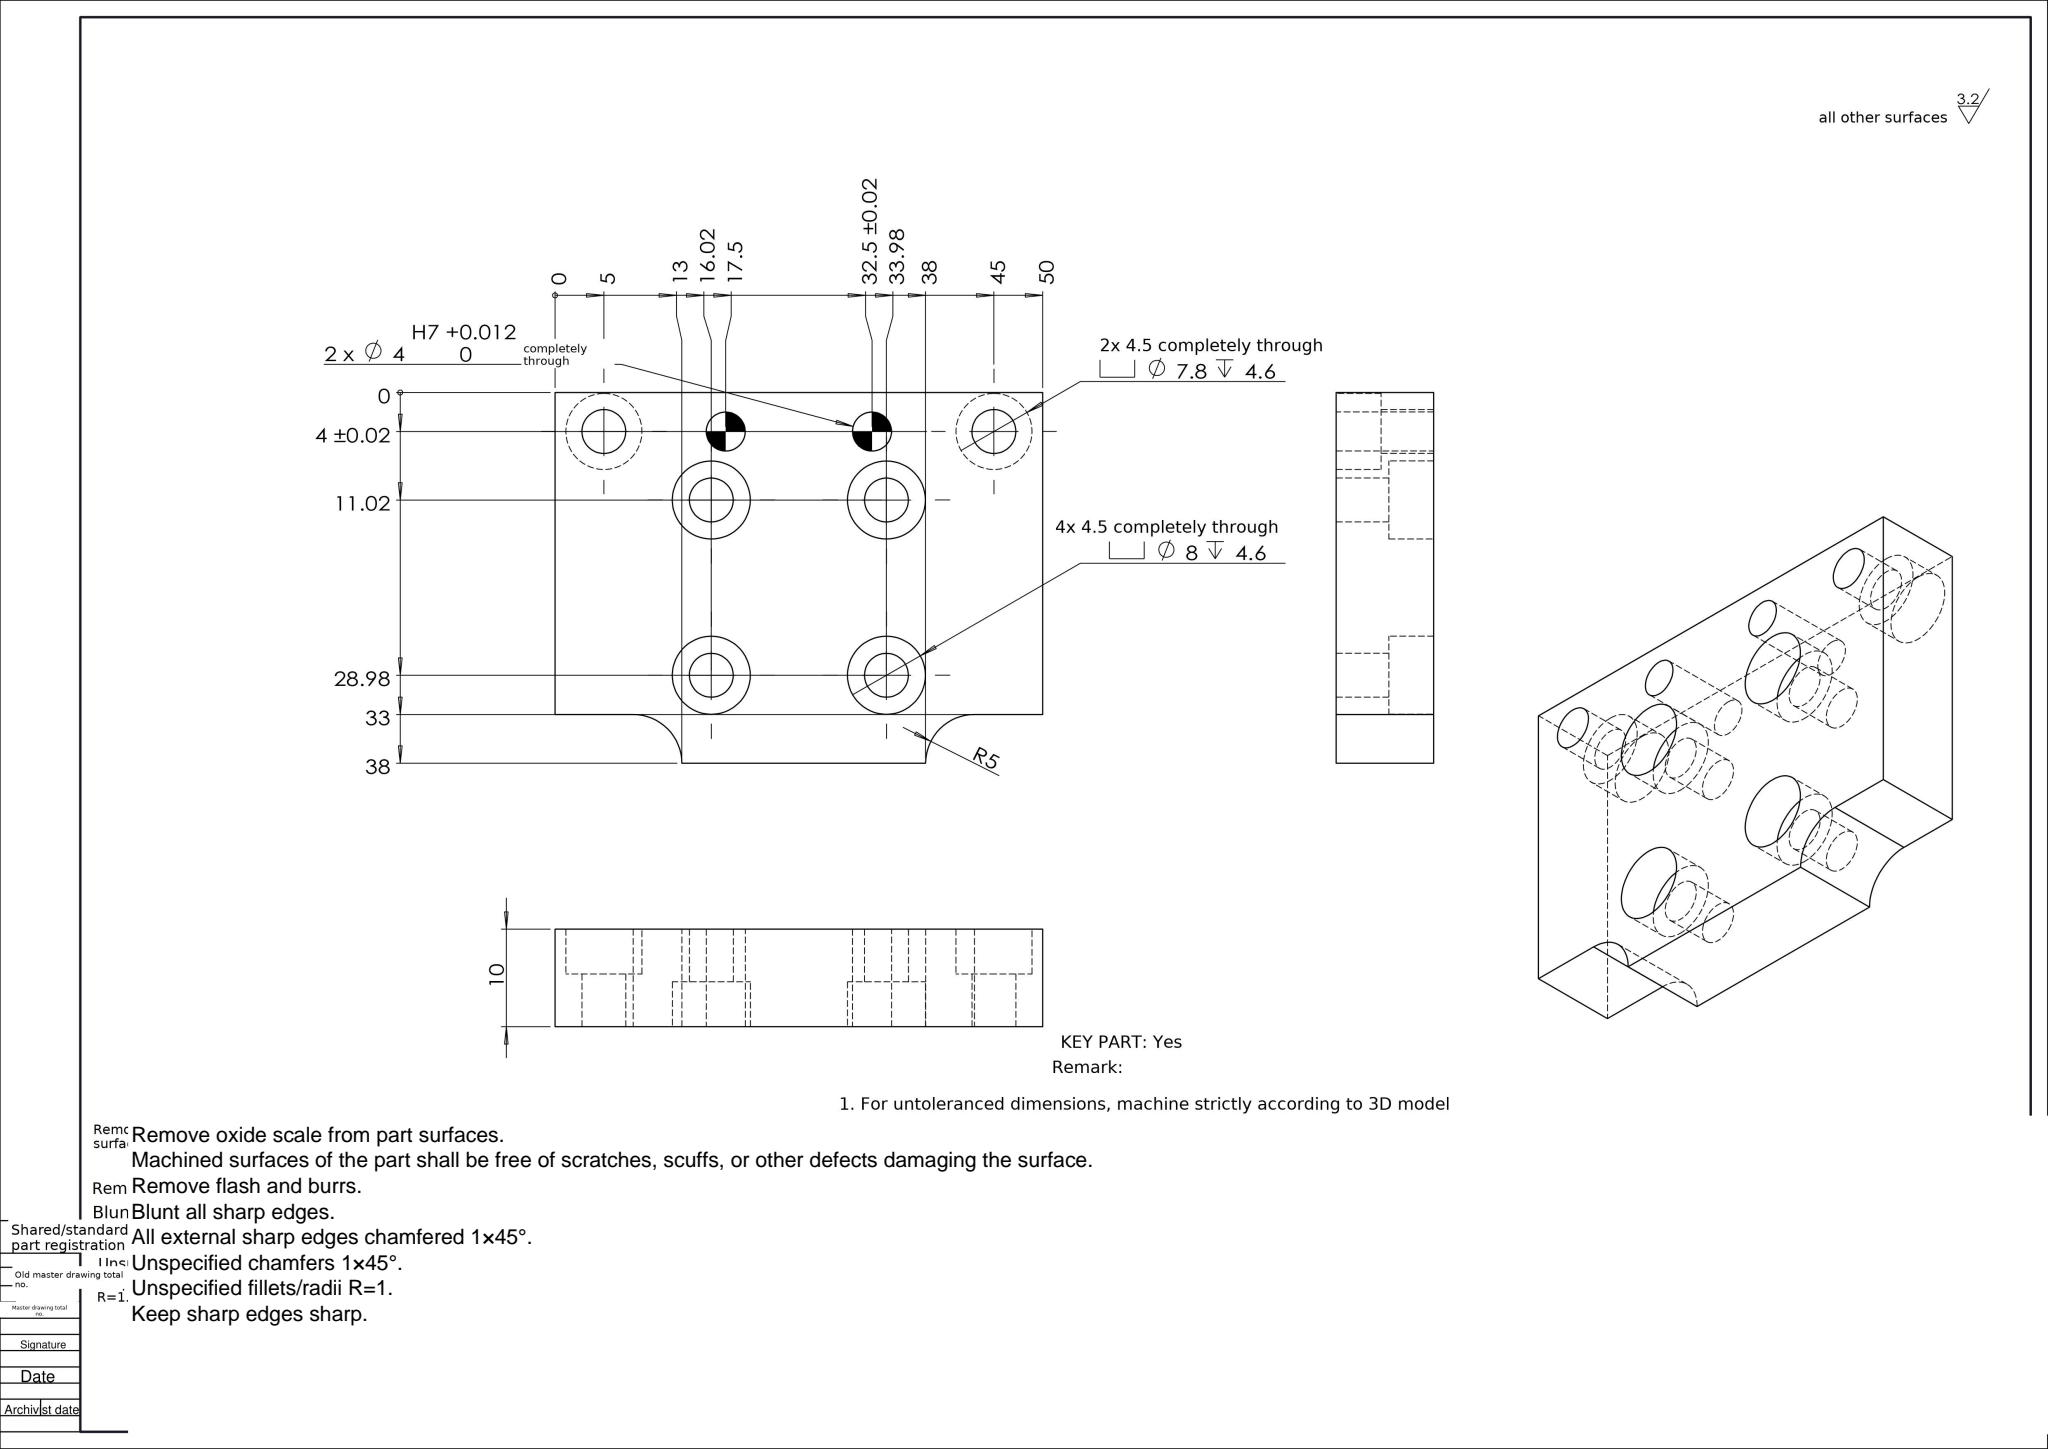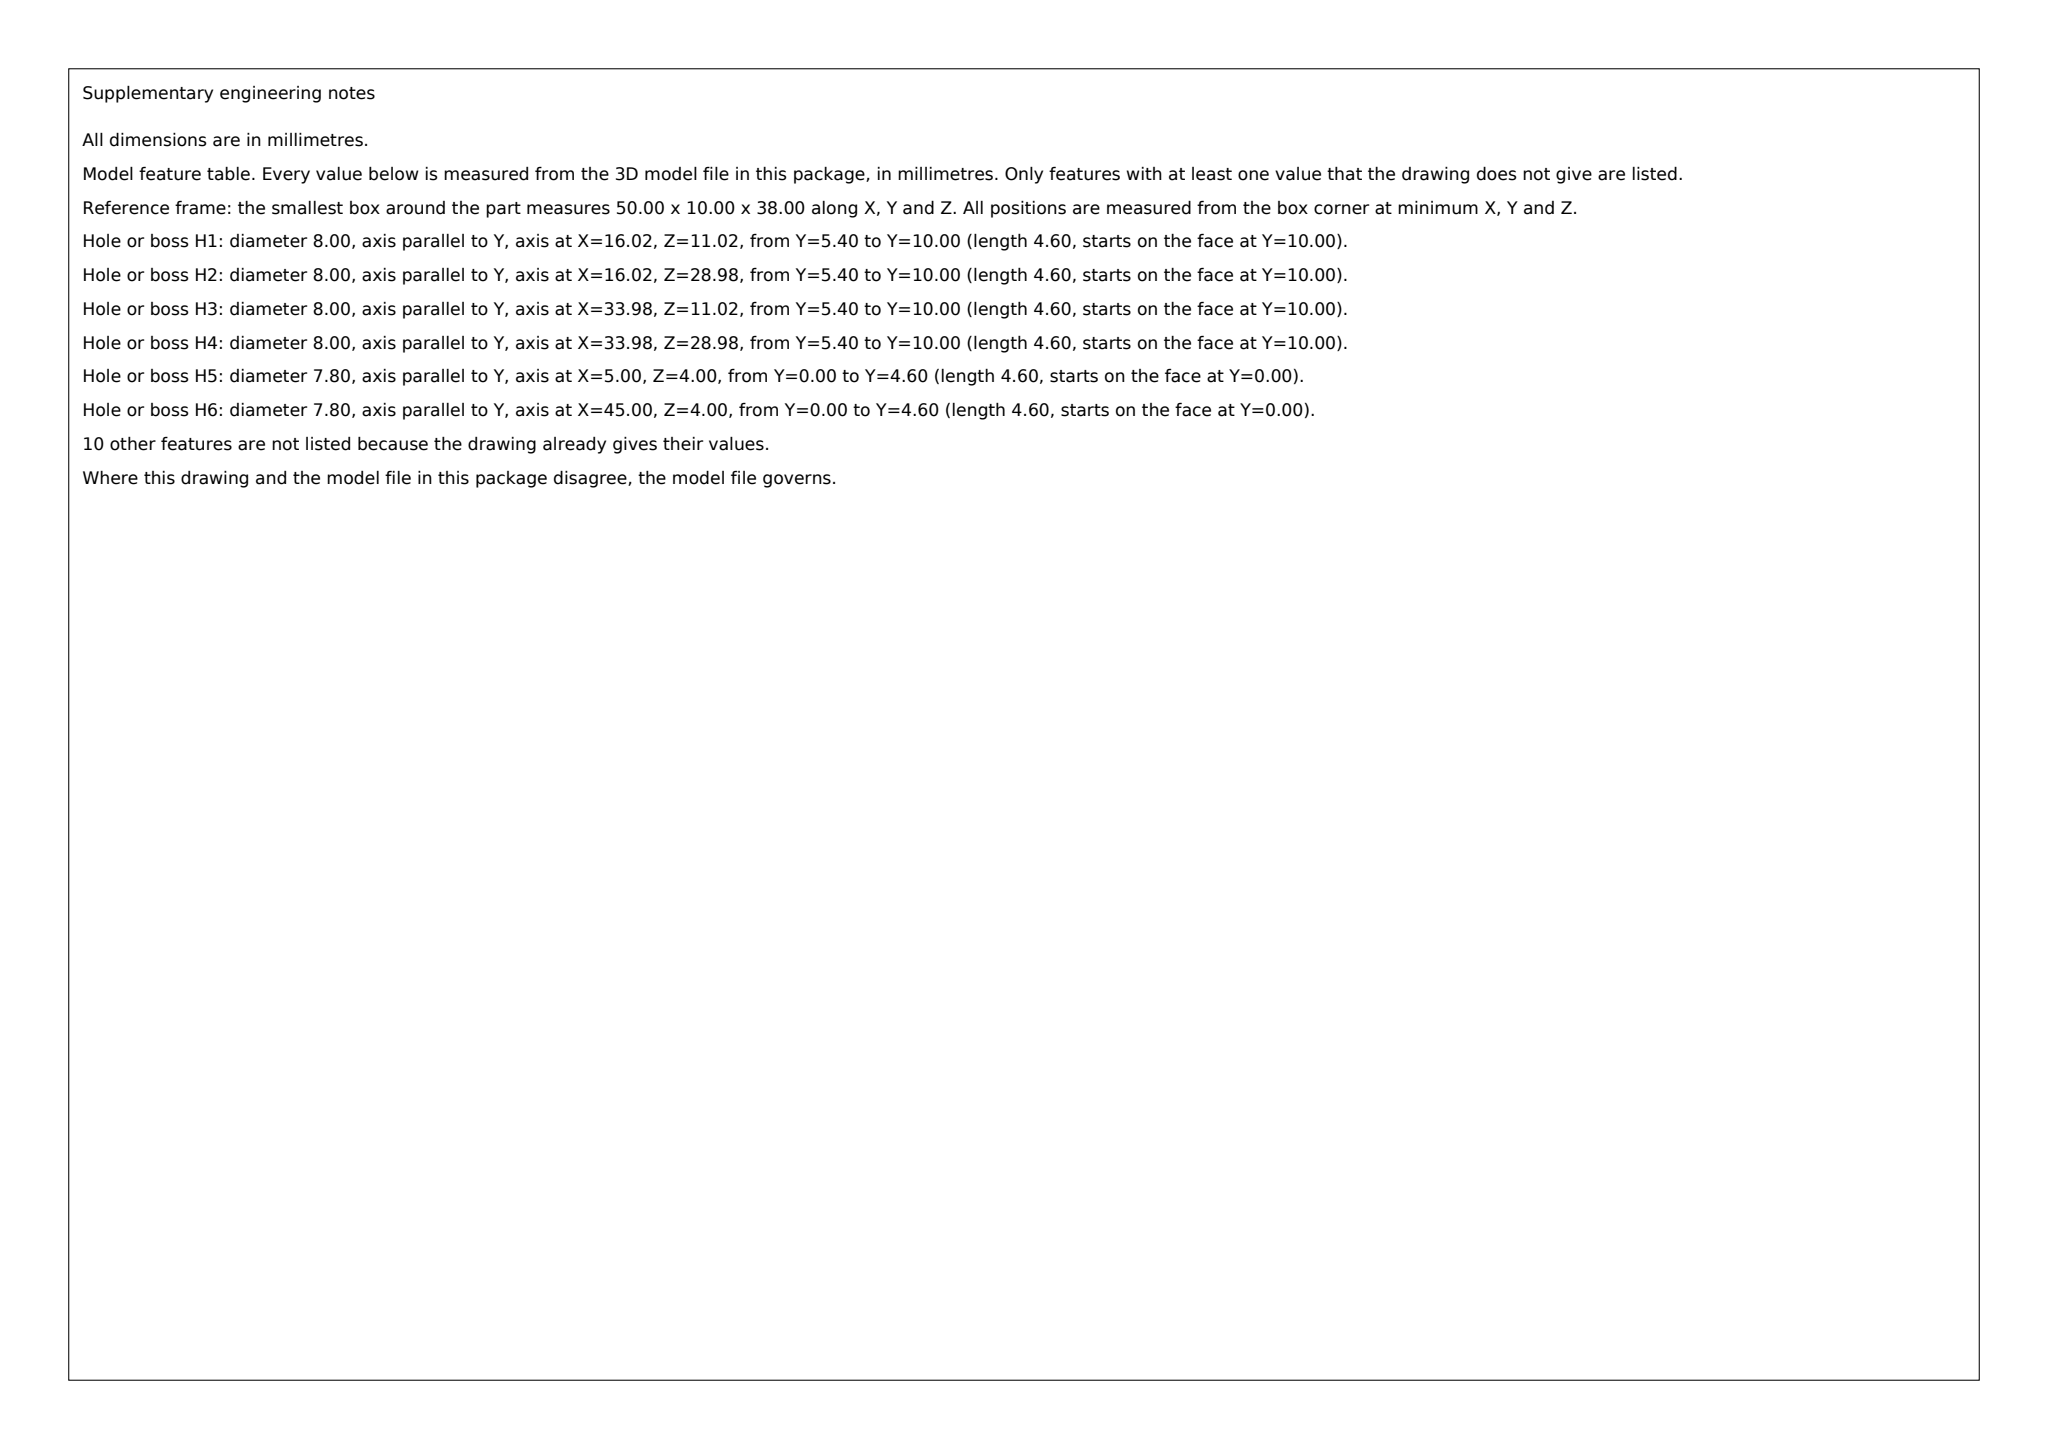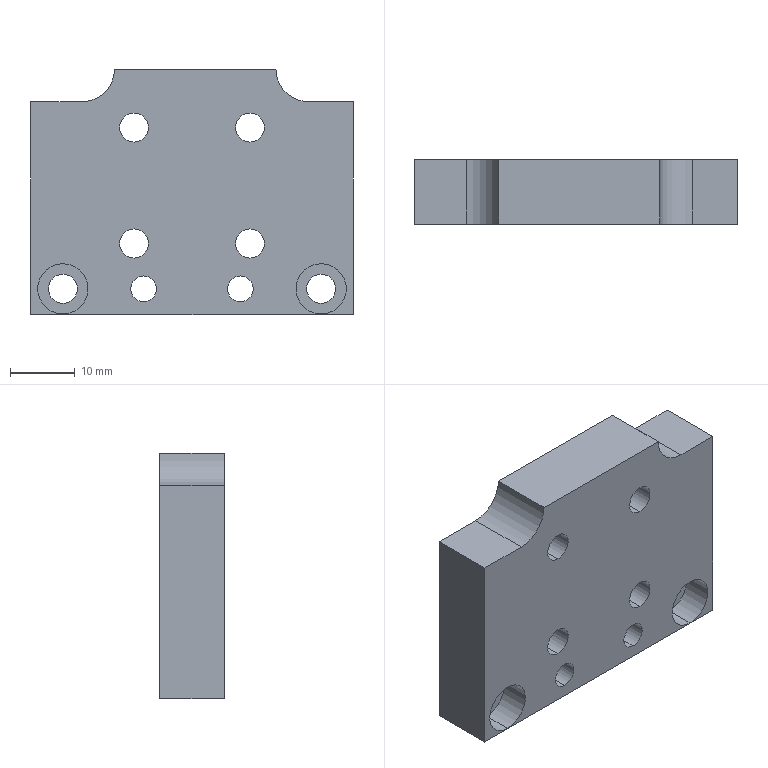Part | SolidWorks | mm | 1 solid | 44 faces | box 50 x 10 x 38 mm | volume 15726 mm3 | cylinder 30 | plane 14 | commonest cylinder face diameters 4.5 x12 8 x8 4 x4 7.8 x4 10 x2